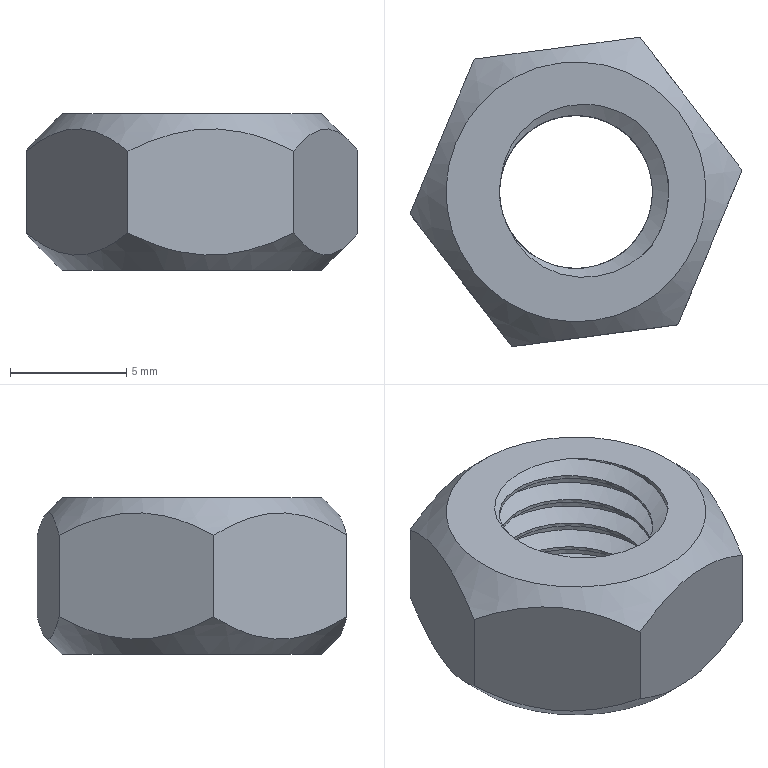Component | NX | NUT | 1 solid | 14 faces | volume 582 mm3 | plane 8 | cone 2 | cylinder 2 | spline 2 | commonest cylinder face diameters 6.6 x1 8 x1